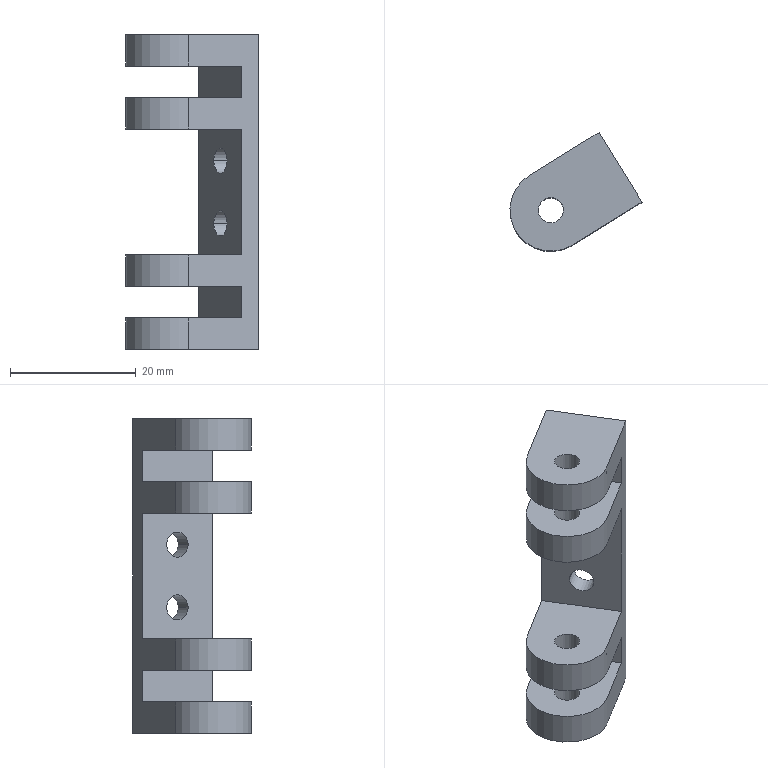Component | SolidWorks | WheelAssembly-1_DamperBase2-1 | 1 solid | 30 faces | box 20.98 x 18.86 x 50 mm | volume 5551 mm3 | cylinder 16 | plane 14 | commonest cylinder face diameters 4 x12 13 x4
build123d program:
from build123d import *

# Parameters (mm, degrees)
SKETCH1_W               = 8
SKETCH1_H               = 8
BOSS_EXTRUDE1_DEPTH     = 42.5
SKETCH2_R               = 2
BOSS_EXTRUDE2_DEPTH     = 25
CUT_EXTRUDE1_DEPTH      = 49.34
CUT_EXTRUDE1_DEPTH_BACK = 49.34
SKETCH3_W               = 5
SKETCH3_H               = 17.65
SKETCH3_W_2             = 20
SKETCH3_H_2             = 17.022
SKETCH4_W               = 50.884
SKETCH4_H               = 95.935
CUT_EXTRUDE2_DEPTH      = 10
SKETCH5_W               = 13
SKETCH5_H               = 50
SKETCH5_R               = 2
BOSS_EXTRUDE3_DEPTH     = 3


with BuildPart() as part:
    # Sketch1 → Boss-Extrude1 (new, symmetric)
    with BuildSketch(Plane.XY):
        Rectangle(SKETCH1_W, SKETCH1_H)
    extrude(amount=BOSS_EXTRUDE1_DEPTH, both=True)

    # Sketch2 → Boss-Extrude2 (add, symmetric)
    with BuildSketch(Plane.XY):
        with BuildLine():
            Line((-6.5, -14), (-6.5, -4))
            Line((-6.5, -4), (6.5, -4))
            Line((6.5, -4), (6.5, -14))
            ThreePointArc((6.5, -14), (0, -20.5), (-6.5, -14))
        make_face()
        with Locations((0, -14)):
            Circle(SKETCH2_R, mode=Mode.SUBTRACT)
    extrude(amount=BOSS_EXTRUDE2_DEPTH, both=True)

    # Sketch3 → Cut-Extrude1 (cut, two sides: drawn at the far end of the back side and taken through both)
    with BuildSketch(Plane(origin=(4, 0, 0), x_dir=(0, 0, -1), z_dir=(1, 0, 0)).offset(-CUT_EXTRUDE1_DEPTH_BACK)):
        with Locations((-17.5, -12.825)):
            Rectangle(SKETCH3_W, SKETCH3_H)
        with Locations((17.5, -12.825)):
            Rectangle(SKETCH3_W, SKETCH3_H)
        with Locations((0, -12.511)):
            Rectangle(SKETCH3_W_2, SKETCH3_H_2)
    extrude(amount=CUT_EXTRUDE1_DEPTH + CUT_EXTRUDE1_DEPTH_BACK, mode=Mode.SUBTRACT)

    # Sketch4 → Cut-Extrude2 (cut)
    with BuildSketch(Plane(origin=(0, -4, 0), x_dir=(1, 0, 0), z_dir=(0, 1, 0))):
        with Locations((5.686, 0.729)):
            Rectangle(SKETCH4_W, SKETCH4_H)
    extrude(amount=CUT_EXTRUDE2_DEPTH, mode=Mode.SUBTRACT)


with BuildPart() as cut_extrude2_piece_1:
    # of the separate pieces the step leaves, piece 1, a body of its own (cut_extrude2_pieces)
    add(part.part.solids().sort_by_distance((-6.5, -4, 15))[0])



with BuildPart() as cut_extrude2_piece_2:
    # of the separate pieces the step leaves, piece 2, a body of its own (cut_extrude2_pieces)
    add(part.part.solids().sort_by_distance((-6.5, -4, -20))[0])


with BuildPart() as cut_extrude2_piece_3:
    # of the separate pieces the step leaves, piece 3, a body of its own (cut_extrude2_pieces)
    add(part.part.solids().sort_by_distance((-6.5, -4, 25))[0])


with BuildPart() as cut_extrude2_piece_4:
    # of the separate pieces the step leaves, piece 4, a body of its own (cut_extrude2_pieces)
    add(part.part.solids().sort_by_distance((-6.5, -4, -10))[0])


with BuildPart() as cut_extrude2_piece_1_1:
    add(cut_extrude2_piece_1.part)

    add(cut_extrude2_piece_2.part)  # Boss-Extrude3 merges Cut-Extrude2 piece 2

    add(cut_extrude2_piece_3.part)  # Boss-Extrude3 merges Cut-Extrude2 piece 3

    add(cut_extrude2_piece_4.part)  # Boss-Extrude3 merges Cut-Extrude2 piece 4
    # Sketch5 → Boss-Extrude3 (add)
    with BuildSketch(Plane(origin=(0, -4, 0), x_dir=(1, 0, 0), z_dir=(0, 1, 0))):
        Rectangle(SKETCH5_W, SKETCH5_H)
        with Locations(Location((0, 5, 0), (0, 0, 180))):
            Circle(SKETCH5_R, mode=Mode.SUBTRACT)
        with Locations(Location((0, -5, 0), (0, 0, 180))):
            Circle(SKETCH5_R, mode=Mode.SUBTRACT)
    extrude(amount=BOSS_EXTRUDE3_DEPTH)


solid = cut_extrude2_piece_1_1.part

# Placed as in the assembly
solid = solid.moved(Location((-246.003, -126.197, -542.97), (0, 0, -58.332)))
STEP:
#1=COLOUR_RGB('',0.7922,0.8196,0.9333);
#2=FILL_AREA_STYLE_COLOUR('',#1);
#3=FILL_AREA_STYLE('',(#2));
#4=SURFACE_STYLE_FILL_AREA(#3);
#5=SURFACE_SIDE_STYLE('',(#4));
#6=SURFACE_STYLE_USAGE(.BOTH.,#5);
#7=PRESENTATION_STYLE_ASSIGNMENT((#6));
#8=CARTESIAN_POINT('',(-10.196,-5.191,-20.983));
#9=VERTEX_POINT('',#8);
#10=CARTESIAN_POINT('',(-10.113,-5.325,-20.983));
#11=VERTEX_POINT('',#10);
#12=CARTESIAN_POINT('',(-10.154,-5.258,-20.983));
#13=DIRECTION('',(0.,0.,1.));
#14=DIRECTION('',(0.8511,0.525,0.));
#15=AXIS2_PLACEMENT_3D('',#12,#13,#14);
#16=CIRCLE('',#15,0.07874);
#17=EDGE_CURVE('',#9,#11,#16,.T.);
#18=ORIENTED_EDGE('',*,*,#17,.F.);
#19=CARTESIAN_POINT('',(-10.196,-5.191,-20.786));
#20=VERTEX_POINT('',#19);
#21=CARTESIAN_POINT('',(-10.196,-5.191,-22.361));
#22=DIRECTION('',(0.,0.,1.));
#23=VECTOR('',#22,39.37);
#24=LINE('',#21,#23);
#25=EDGE_CURVE('',#9,#20,#24,.T.);
#26=ORIENTED_EDGE('',*,*,#25,.T.);
#27=CARTESIAN_POINT('',(-10.113,-5.325,-20.786));
#28=VERTEX_POINT('',#27);
#29=CARTESIAN_POINT('',(-10.154,-5.258,-20.786));
#30=DIRECTION('',(-0.,-0.,-1.));
#31=DIRECTION('',(-0.8511,-0.525,0.));
#32=AXIS2_PLACEMENT_3D('',#29,#30,#31);
#33=CIRCLE('',#32,0.07874);
#34=EDGE_CURVE('',#28,#20,#33,.T.);
#35=ORIENTED_EDGE('',*,*,#34,.F.);
#36=CARTESIAN_POINT('',(-10.113,-5.325,-22.361));
#37=DIRECTION('',(0.,0.,1.));
#38=VECTOR('',#37,39.37);
#39=LINE('',#36,#38);
#40=EDGE_CURVE('',#11,#28,#39,.T.);
#41=ORIENTED_EDGE('',*,*,#40,.F.);
#42=EDGE_LOOP('',(#18,#26,#35,#41));
#43=FACE_OUTER_BOUND('',#42,.T.);
#44=CARTESIAN_POINT('',(-10.154,-5.258,-22.361));
#45=DIRECTION('',(0.,0.,1.));
#46=DIRECTION('',(0.525,-0.8511,0.));
#47=AXIS2_PLACEMENT_3D('',#44,#45,#46);
#48=CYLINDRICAL_SURFACE('',#47,0.07874);
#49=ADVANCED_FACE('',(#43),#48,.F.);
#50=CARTESIAN_POINT('',(-10.196,-5.191,-20.589));
#51=VERTEX_POINT('',#50);
#52=CARTESIAN_POINT('',(-10.113,-5.325,-20.589));
#53=VERTEX_POINT('',#52);
#54=CARTESIAN_POINT('',(-10.154,-5.258,-20.589));
#55=DIRECTION('',(0.,0.,1.));
#56=DIRECTION('',(0.8511,0.525,0.));
#57=AXIS2_PLACEMENT_3D('',#54,#55,#56);
#58=CIRCLE('',#57,0.07874);
#59=EDGE_CURVE('',#51,#53,#58,.T.);
#60=ORIENTED_EDGE('',*,*,#59,.F.);
#61=CARTESIAN_POINT('',(-10.196,-5.191,-20.393));
#62=VERTEX_POINT('',#61);
#63=CARTESIAN_POINT('',(-10.196,-5.191,-22.361));
#64=DIRECTION('',(0.,0.,1.));
#65=VECTOR('',#64,39.37);
#66=LINE('',#63,#65);
#67=EDGE_CURVE('',#51,#62,#66,.T.);
#68=ORIENTED_EDGE('',*,*,#67,.T.);
#69=CARTESIAN_POINT('',(-10.113,-5.325,-20.393));
#70=VERTEX_POINT('',#69);
#71=CARTESIAN_POINT('',(-10.154,-5.258,-20.393));
#72=DIRECTION('',(-0.,-0.,-1.));
#73=DIRECTION('',(-0.525,0.8511,-0.));
#74=AXIS2_PLACEMENT_3D('',#71,#72,#73);
#75=CIRCLE('',#74,0.07874);
#76=EDGE_CURVE('',#70,#62,#75,.T.);
#77=ORIENTED_EDGE('',*,*,#76,.F.);
#78=CARTESIAN_POINT('',(-10.113,-5.325,-22.361));
#79=DIRECTION('',(0.,0.,1.));
#80=VECTOR('',#79,39.37);
#81=LINE('',#78,#80);
#82=EDGE_CURVE('',#53,#70,#81,.T.);
#83=ORIENTED_EDGE('',*,*,#82,.F.);
#84=EDGE_LOOP('',(#60,#68,#77,#83));
#85=FACE_OUTER_BOUND('',#84,.T.);
#86=CARTESIAN_POINT('',(-10.154,-5.258,-22.361));
#87=DIRECTION('',(0.,0.,1.));
#88=DIRECTION('',(0.525,-0.8511,0.));
#89=AXIS2_PLACEMENT_3D('',#86,#87,#88);
#90=CYLINDRICAL_SURFACE('',#89,0.07874);
#91=ADVANCED_FACE('',(#85),#90,.F.);
#92=CARTESIAN_POINT('',(-10.196,-5.191,-21.967));
#93=VERTEX_POINT('',#92);
#94=CARTESIAN_POINT('',(-10.113,-5.325,-21.967));
#95=VERTEX_POINT('',#94);
#96=CARTESIAN_POINT('',(-10.154,-5.258,-21.967));
#97=DIRECTION('',(0.,0.,1.));
#98=DIRECTION('',(0.8511,0.525,0.));
#99=AXIS2_PLACEMENT_3D('',#96,#97,#98);
#100=CIRCLE('',#99,0.07874);
#101=EDGE_CURVE('',#93,#95,#100,.T.);
#102=ORIENTED_EDGE('',*,*,#101,.F.);
#103=CARTESIAN_POINT('',(-10.196,-5.191,-21.77));
#104=VERTEX_POINT('',#103);
#105=CARTESIAN_POINT('',(-10.196,-5.191,-22.361));
#106=DIRECTION('',(0.,0.,1.));
#107=VECTOR('',#106,39.37);
#108=LINE('',#105,#107);
#109=EDGE_CURVE('',#93,#104,#108,.T.);
#110=ORIENTED_EDGE('',*,*,#109,.T.);
#111=CARTESIAN_POINT('',(-10.113,-5.325,-21.77));
#112=VERTEX_POINT('',#111);
#113=CARTESIAN_POINT('',(-10.154,-5.258,-21.77));
#114=DIRECTION('',(-0.,-0.,-1.));
#115=DIRECTION('',(-0.8511,-0.525,0.));
#116=AXIS2_PLACEMENT_3D('',#113,#114,#115);
#117=CIRCLE('',#116,0.07874);
#118=EDGE_CURVE('',#112,#104,#117,.T.);
#119=ORIENTED_EDGE('',*,*,#118,.F.);
#120=CARTESIAN_POINT('',(-10.113,-5.325,-22.361));
#121=DIRECTION('',(0.,0.,1.));
#122=VECTOR('',#121,39.37);
#123=LINE('',#120,#122);
#124=EDGE_CURVE('',#95,#112,#123,.T.);
#125=ORIENTED_EDGE('',*,*,#124,.F.);
#126=EDGE_LOOP('',(#102,#110,#119,#125));
#127=FACE_OUTER_BOUND('',#126,.T.);
#128=CARTESIAN_POINT('',(-10.154,-5.258,-22.361));
#129=DIRECTION('',(0.,0.,1.));
#130=DIRECTION('',(0.525,-0.8511,0.));
#131=AXIS2_PLACEMENT_3D('',#128,#129,#130);
#132=CYLINDRICAL_SURFACE('',#131,0.07874);
#133=ADVANCED_FACE('',(#127),#132,.F.);
#134=CARTESIAN_POINT('',(-9.76,-4.922,-21.574));
#135=VERTEX_POINT('',#134);
#136=CARTESIAN_POINT('',(-9.677,-5.056,-21.574));
#137=VERTEX_POINT('',#136);
#138=CARTESIAN_POINT('',(-9.719,-4.989,-21.574));
#139=DIRECTION('',(0.8511,0.525,-0.));
#140=DIRECTION('',(0.525,-0.8511,0.));
#141=AXIS2_PLACEMENT_3D('',#138,#139,#140);
#142=CIRCLE('',#141,0.07874);
#143=EDGE_CURVE('',#135,#137,#142,.T.);
#144=ORIENTED_EDGE('',*,*,#143,.T.);
#145=CARTESIAN_POINT('',(-9.778,-5.118,-21.574));
#146=VERTEX_POINT('',#145);
#147=CARTESIAN_POINT('',(-9.677,-5.056,-21.574));
#148=DIRECTION('',(-0.8511,-0.525,0.));
#149=VECTOR('',#148,39.37);
#150=LINE('',#147,#149);
#151=EDGE_CURVE('',#137,#146,#150,.T.);
#152=ORIENTED_EDGE('',*,*,#151,.T.);
#153=CARTESIAN_POINT('',(-9.861,-4.984,-21.574));
#154=VERTEX_POINT('',#153);
#155=CARTESIAN_POINT('',(-9.819,-5.051,-21.574));
#156=DIRECTION('',(0.8511,0.525,-0.));
#157=DIRECTION('',(0.525,-0.8511,0.));
#158=AXIS2_PLACEMENT_3D('',#155,#156,#157);
#159=CIRCLE('',#158,0.07874);
#160=EDGE_CURVE('',#154,#146,#159,.T.);
#161=ORIENTED_EDGE('',*,*,#160,.F.);
#162=CARTESIAN_POINT('',(-9.76,-4.922,-21.574));
#163=DIRECTION('',(-0.8511,-0.525,0.));
#164=VECTOR('',#163,39.37);
#165=LINE('',#162,#164);
#166=EDGE_CURVE('',#135,#154,#165,.T.);
#167=ORIENTED_EDGE('',*,*,#166,.F.);
#168=EDGE_LOOP('',(#144,#152,#161,#167));
#169=FACE_OUTER_BOUND('',#168,.T.);
#170=CARTESIAN_POINT('',(-9.719,-4.989,-21.574));
#171=DIRECTION('',(-0.8511,-0.525,0.));
#172=DIRECTION('',(-0.525,0.8511,-0.));
#173=AXIS2_PLACEMENT_3D('',#170,#171,#172);
#174=CYLINDRICAL_SURFACE('',#173,0.07874);
#175=ADVANCED_FACE('',(#169),#174,.F.);
#176=CARTESIAN_POINT('',(-9.76,-4.922,-21.18));
#177=VERTEX_POINT('',#176);
#178=CARTESIAN_POINT('',(-9.677,-5.056,-21.18));
#179=VERTEX_POINT('',#178);
#180=CARTESIAN_POINT('',(-9.719,-4.989,-21.18));
#181=DIRECTION('',(0.8511,0.525,-0.));
#182=DIRECTION('',(0.525,-0.8511,0.));
#183=AXIS2_PLACEMENT_3D('',#180,#181,#182);
#184=CIRCLE('',#183,0.07874);
#185=EDGE_CURVE('',#177,#179,#184,.T.);
#186=ORIENTED_EDGE('',*,*,#185,.T.);
#187=CARTESIAN_POINT('',(-9.778,-5.118,-21.18));
#188=VERTEX_POINT('',#187);
#189=CARTESIAN_POINT('',(-9.677,-5.056,-21.18));
#190=DIRECTION('',(-0.8511,-0.525,0.));
#191=VECTOR('',#190,39.37);
#192=LINE('',#189,#191);
#193=EDGE_CURVE('',#179,#188,#192,.T.);
#194=ORIENTED_EDGE('',*,*,#193,.T.);
#195=CARTESIAN_POINT('',(-9.861,-4.984,-21.18));
#196=VERTEX_POINT('',#195);
#197=CARTESIAN_POINT('',(-9.819,-5.051,-21.18));
#198=DIRECTION('',(0.8511,0.525,-0.));
#199=DIRECTION('',(0.525,-0.8511,0.));
#200=AXIS2_PLACEMENT_3D('',#197,#198,#199);
#201=CIRCLE('',#200,0.07874);
#202=EDGE_CURVE('',#196,#188,#201,.T.);
#203=ORIENTED_EDGE('',*,*,#202,.F.);
#204=CARTESIAN_POINT('',(-9.76,-4.922,-21.18));
#205=DIRECTION('',(-0.8511,-0.525,0.));
#206=VECTOR('',#205,39.37);
#207=LINE('',#204,#206);
#208=EDGE_CURVE('',#177,#196,#207,.T.);
#209=ORIENTED_EDGE('',*,*,#208,.F.);
#210=EDGE_LOOP('',(#186,#194,#203,#209));
#211=FACE_OUTER_BOUND('',#210,.T.);
#212=CARTESIAN_POINT('',(-9.719,-4.989,-21.18));
#213=DIRECTION('',(-0.8511,-0.525,0.));
#214=DIRECTION('',(-0.525,0.8511,-0.));
#215=AXIS2_PLACEMENT_3D('',#212,#213,#214);
#216=CYLINDRICAL_SURFACE('',#215,0.07874);
#217=ADVANCED_FACE('',(#211),#216,.F.);
#218=CARTESIAN_POINT('',(-10.113,-5.325,-22.361));
#219=VERTEX_POINT('',#218);
#220=CARTESIAN_POINT('',(-10.196,-5.191,-22.361));
#221=VERTEX_POINT('',#220);
#222=CARTESIAN_POINT('',(-10.154,-5.258,-22.361));
#223=DIRECTION('',(-0.,-0.,-1.));
#224=DIRECTION('',(-0.525,0.8511,-0.));
#225=AXIS2_PLACEMENT_3D('',#222,#223,#224);
#226=CIRCLE('',#225,0.07874);
#227=EDGE_CURVE('',#219,#221,#226,.T.);
#228=ORIENTED_EDGE('',*,*,#227,.T.);
#229=CARTESIAN_POINT('',(-10.196,-5.191,-22.164));
#230=VERTEX_POINT('',#229);
#231=CARTESIAN_POINT('',(-10.196,-5.191,-22.361));
#232=DIRECTION('',(0.,0.,1.));
#233=VECTOR('',#232,39.37);
#234=LINE('',#231,#233);
#235=EDGE_CURVE('',#221,#230,#234,.T.);
#236=ORIENTED_EDGE('',*,*,#235,.T.);
#237=CARTESIAN_POINT('',(-10.113,-5.325,-22.164));
#238=VERTEX_POINT('',#237);
#239=CARTESIAN_POINT('',(-10.154,-5.258,-22.164));
#240=DIRECTION('',(-0.,-0.,-1.));
#241=DIRECTION('',(-0.8511,-0.525,0.));
#242=AXIS2_PLACEMENT_3D('',#239,#240,#241);
#243=CIRCLE('',#242,0.07874);
#244=EDGE_CURVE('',#238,#230,#243,.T.);
#245=ORIENTED_EDGE('',*,*,#244,.F.);
#246=CARTESIAN_POINT('',(-10.113,-5.325,-22.361));
#247=DIRECTION('',(0.,0.,1.));
#248=VECTOR('',#247,39.37);
#249=LINE('',#246,#248);
#250=EDGE_CURVE('',#219,#238,#249,.T.);
#251=ORIENTED_EDGE('',*,*,#250,.F.);
#252=EDGE_LOOP('',(#228,#236,#245,#251));
#253=FACE_OUTER_BOUND('',#252,.T.);
#254=CARTESIAN_POINT('',(-10.154,-5.258,-22.361));
#255=DIRECTION('',(0.,0.,1.));
#256=DIRECTION('',(0.525,-0.8511,0.));
#257=AXIS2_PLACEMENT_3D('',#254,#255,#256);
#258=CYLINDRICAL_SURFACE('',#257,0.07874);
#259=ADVANCED_FACE('',(#253),#258,.F.);
#260=ORIENTED_EDGE('',*,*,#160,.T.);
#261=CARTESIAN_POINT('',(-9.819,-5.051,-21.574));
#262=DIRECTION('',(0.8511,0.525,-0.));
#263=DIRECTION('',(0.525,-0.8511,0.));
#264=AXIS2_PLACEMENT_3D('',#261,#262,#263);
#265=CIRCLE('',#264,0.07874);
#266=EDGE_CURVE('',#146,#154,#265,.T.);
#267=ORIENTED_EDGE('',*,*,#266,.T.);
#268=EDGE_LOOP('',(#260,#267));
#269=FACE_BOUND('',#268,.T.);
#270=ORIENTED_EDGE('',*,*,#202,.T.);
#271=CARTESIAN_POINT('',(-9.819,-5.051,-21.18));
#272=DIRECTION('',(0.8511,0.525,-0.));
#273=DIRECTION('',(0.525,-0.8511,0.));
#274=AXIS2_PLACEMENT_3D('',#271,#272,#273);
#275=CIRCLE('',#274,0.07874);
#276=EDGE_CURVE('',#188,#196,#275,.T.);
#277=ORIENTED_EDGE('',*,*,#276,.T.);
#278=EDGE_LOOP('',(#270,#277));
#279=FACE_BOUND('',#278,.T.);
#280=CARTESIAN_POINT('',(-9.685,-5.269,-20.983));
#281=VERTEX_POINT('',#280);
#282=CARTESIAN_POINT('',(-9.954,-4.833,-20.983));
#283=VERTEX_POINT('',#282);
#284=CARTESIAN_POINT('',(-9.685,-5.269,-20.983));
#285=DIRECTION('',(-0.525,0.8511,-0.));
#286=VECTOR('',#285,39.37);
#287=LINE('',#284,#286);
#288=EDGE_CURVE('',#281,#283,#287,.T.);
#289=ORIENTED_EDGE('',*,*,#288,.T.);
#290=CARTESIAN_POINT('',(-9.954,-4.833,-21.77));
#291=VERTEX_POINT('',#290);
#292=CARTESIAN_POINT('',(-9.954,-4.833,-20.393));
#293=DIRECTION('',(0.,0.,1.));
#294=VECTOR('',#293,39.37);
#295=LINE('',#292,#294);
#296=EDGE_CURVE('',#291,#283,#295,.T.);
#297=ORIENTED_EDGE('',*,*,#296,.F.);
#298=CARTESIAN_POINT('',(-9.685,-5.269,-21.77));
#299=VERTEX_POINT('',#298);
#300=CARTESIAN_POINT('',(-9.685,-5.269,-21.77));
#301=DIRECTION('',(-0.525,0.8511,-0.));
#302=VECTOR('',#301,39.37);
#303=LINE('',#300,#302);
#304=EDGE_CURVE('',#299,#291,#303,.T.);
#305=ORIENTED_EDGE('',*,*,#304,.F.);
#306=CARTESIAN_POINT('',(-9.685,-5.269,-20.393));
#307=DIRECTION('',(-0.,-0.,-1.));
#308=VECTOR('',#307,39.37);
#309=LINE('',#306,#308);
#310=EDGE_CURVE('',#281,#299,#309,.T.);
#311=ORIENTED_EDGE('',*,*,#310,.F.);
#312=EDGE_LOOP('',(#289,#297,#305,#311));
#313=FACE_OUTER_BOUND('',#312,.T.);
#314=CARTESIAN_POINT('',(-9.819,-5.051,-21.377));
#315=DIRECTION('',(0.8511,0.525,-0.));
#316=DIRECTION('',(-0.,-0.,-1.));
#317=AXIS2_PLACEMENT_3D('',#314,#315,#316);
#318=PLANE('',#317);
#319=ADVANCED_FACE('',(#269,#279,#313),#318,.F.);
#320=CARTESIAN_POINT('',(-9.685,-5.269,-20.786));
#321=VERTEX_POINT('',#320);
#322=CARTESIAN_POINT('',(-9.954,-4.833,-20.786));
#323=VERTEX_POINT('',#322);
#324=CARTESIAN_POINT('',(-9.685,-5.269,-20.786));
#325=DIRECTION('',(-0.525,0.8511,-0.));
#326=VECTOR('',#325,39.37);
#327=LINE('',#324,#326);
#328=EDGE_CURVE('',#321,#323,#327,.T.);
#329=ORIENTED_EDGE('',*,*,#328,.F.);
#330=CARTESIAN_POINT('',(-9.685,-5.269,-20.589));
#331=VERTEX_POINT('',#330);
#332=CARTESIAN_POINT('',(-9.685,-5.269,-20.393));
#333=DIRECTION('',(-0.,-0.,-1.));
#334=VECTOR('',#333,39.37);
#335=LINE('',#332,#334);
#336=EDGE_CURVE('',#331,#321,#335,.T.);
#337=ORIENTED_EDGE('',*,*,#336,.F.);
#338=CARTESIAN_POINT('',(-9.954,-4.833,-20.589));
#339=VERTEX_POINT('',#338);
#340=CARTESIAN_POINT('',(-9.685,-5.269,-20.589));
#341=DIRECTION('',(-0.525,0.8511,-0.));
#342=VECTOR('',#341,39.37);
#343=LINE('',#340,#342);
#344=EDGE_CURVE('',#331,#339,#343,.T.);
#345=ORIENTED_EDGE('',*,*,#344,.T.);
#346=CARTESIAN_POINT('',(-9.954,-4.833,-20.393));
#347=DIRECTION('',(0.,0.,1.));
#348=VECTOR('',#347,39.37);
#349=LINE('',#346,#348);
#350=EDGE_CURVE('',#323,#339,#349,.T.);
#351=ORIENTED_EDGE('',*,*,#350,.F.);
#352=EDGE_LOOP('',(#329,#337,#345,#351));
#353=FACE_OUTER_BOUND('',#352,.T.);
#354=CARTESIAN_POINT('',(-9.819,-5.051,-21.377));
#355=DIRECTION('',(0.8511,0.525,-0.));
#356=DIRECTION('',(-0.,-0.,-1.));
#357=AXIS2_PLACEMENT_3D('',#354,#355,#356);
#358=PLANE('',#357);
#359=ADVANCED_FACE('',(#353),#358,.F.);
#360=CARTESIAN_POINT('',(-9.685,-5.269,-21.967));
#361=VERTEX_POINT('',#360);
#362=CARTESIAN_POINT('',(-9.954,-4.833,-21.967));
#363=VERTEX_POINT('',#362);
#364=CARTESIAN_POINT('',(-9.685,-5.269,-21.967));
#365=DIRECTION('',(-0.525,0.8511,-0.));
#366=VECTOR('',#365,39.37);
#367=LINE('',#364,#366);
#368=EDGE_CURVE('',#361,#363,#367,.T.);
#369=ORIENTED_EDGE('',*,*,#368,.T.);
#370=CARTESIAN_POINT('',(-9.954,-4.833,-22.164));
#371=VERTEX_POINT('',#370);
#372=CARTESIAN_POINT('',(-9.954,-4.833,-20.393));
#373=DIRECTION('',(0.,0.,1.));
#374=VECTOR('',#373,39.37);
#375=LINE('',#372,#374);
#376=EDGE_CURVE('',#371,#363,#375,.T.);
#377=ORIENTED_EDGE('',*,*,#376,.F.);
#378=CARTESIAN_POINT('',(-9.685,-5.269,-22.164));
#379=VERTEX_POINT('',#378);
#380=CARTESIAN_POINT('',(-9.685,-5.269,-22.164));
#381=DIRECTION('',(-0.525,0.8511,-0.));
#382=VECTOR('',#381,39.37);
#383=LINE('',#380,#382);
#384=EDGE_CURVE('',#379,#371,#383,.T.);
#385=ORIENTED_EDGE('',*,*,#384,.F.);
#386=CARTESIAN_POINT('',(-9.685,-5.269,-20.393));
#387=DIRECTION('',(-0.,-0.,-1.));
#388=VECTOR('',#387,39.37);
#389=LINE('',#386,#388);
#390=EDGE_CURVE('',#361,#379,#389,.T.);
#391=ORIENTED_EDGE('',*,*,#390,.F.);
#392=EDGE_LOOP('',(#369,#377,#385,#391));
#393=FACE_OUTER_BOUND('',#392,.T.);
#394=CARTESIAN_POINT('',(-9.819,-5.051,-21.377));
#395=DIRECTION('',(0.8511,0.525,-0.));
#396=DIRECTION('',(-0.,-0.,-1.));
#397=AXIS2_PLACEMENT_3D('',#394,#395,#396);
#398=PLANE('',#397);
#399=ADVANCED_FACE('',(#393),#398,.F.);
#400=CARTESIAN_POINT('',(-10.02,-5.476,-22.361));
#401=VERTEX_POINT('',#400);
#402=CARTESIAN_POINT('',(-10.02,-5.476,-22.164));
#403=VERTEX_POINT('',#402);
#404=CARTESIAN_POINT('',(-10.02,-5.476,-22.361));
#405=DIRECTION('',(0.,0.,1.));
#406=VECTOR('',#405,39.37);
#407=LINE('',#404,#406);
#408=EDGE_CURVE('',#401,#403,#407,.T.);
#409=ORIENTED_EDGE('',*,*,#408,.T.);
#410=CARTESIAN_POINT('',(-10.289,-5.04,-22.164));
#411=VERTEX_POINT('',#410);
#412=CARTESIAN_POINT('',(-10.154,-5.258,-22.164));
#413=DIRECTION('',(-0.,-0.,-1.));
#414=DIRECTION('',(-0.8511,-0.525,0.));
#415=AXIS2_PLACEMENT_3D('',#412,#413,#414);
#416=CIRCLE('',#415,0.2559);
#417=EDGE_CURVE('',#403,#411,#416,.T.);
#418=ORIENTED_EDGE('',*,*,#417,.T.);
#419=CARTESIAN_POINT('',(-10.289,-5.04,-22.361));
#420=VERTEX_POINT('',#419);
#421=CARTESIAN_POINT('',(-10.289,-5.04,-22.361));
#422=DIRECTION('',(0.,0.,1.));
#423=VECTOR('',#422,39.37);
#424=LINE('',#421,#423);
#425=EDGE_CURVE('',#420,#411,#424,.T.);
#426=ORIENTED_EDGE('',*,*,#425,.F.);
#427=CARTESIAN_POINT('',(-10.154,-5.258,-22.361));
#428=DIRECTION('',(-0.,-0.,-1.));
#429=DIRECTION('',(-0.525,0.8511,-0.));
#430=AXIS2_PLACEMENT_3D('',#427,#428,#429);
#431=CIRCLE('',#430,0.2559);
#432=EDGE_CURVE('',#401,#420,#431,.T.);
#433=ORIENTED_EDGE('',*,*,#432,.F.);
#434=EDGE_LOOP('',(#409,#418,#426,#433));
#435=FACE_OUTER_BOUND('',#434,.T.);
#436=CARTESIAN_POINT('',(-10.154,-5.258,-22.361));
#437=DIRECTION('',(0.,0.,1.));
#438=DIRECTION('',(0.525,-0.8511,0.));
#439=AXIS2_PLACEMENT_3D('',#436,#437,#438);
#440=CYLINDRICAL_SURFACE('',#439,0.2559);
#441=ADVANCED_FACE('',(#435),#440,.T.);
#442=ORIENTED_EDGE('',*,*,#425,.T.);
#443=CARTESIAN_POINT('',(-9.954,-4.833,-22.164));
#444=DIRECTION('',(-0.8511,-0.525,0.));
#445=VECTOR('',#444,39.37);
#446=LINE('',#443,#445);
#447=EDGE_CURVE('',#371,#411,#446,.T.);
#448=ORIENTED_EDGE('',*,*,#447,.F.);
#449=ORIENTED_EDGE('',*,*,#376,.T.);
#450=CARTESIAN_POINT('',(-10.289,-5.04,-21.967));
#451=VERTEX_POINT('',#450);
#452=CARTESIAN_POINT('',(-9.954,-4.833,-21.967));
#453=DIRECTION('',(0.8511,0.525,-0.));
#454=VECTOR('',#453,39.37);
#455=LINE('',#452,#454);
#456=EDGE_CURVE('',#451,#363,#455,.T.);
#457=ORIENTED_EDGE('',*,*,#456,.F.);
#458=CARTESIAN_POINT('',(-10.289,-5.04,-21.77));
#459=VERTEX_POINT('',#458);
#460=CARTESIAN_POINT('',(-10.289,-5.04,-22.361));
#461=DIRECTION('',(0.,0.,1.));
#462=VECTOR('',#461,39.37);
#463=LINE('',#460,#462);
#464=EDGE_CURVE('',#451,#459,#463,.T.);
#465=ORIENTED_EDGE('',*,*,#464,.T.);
#466=CARTESIAN_POINT('',(-9.954,-4.833,-21.77));
#467=DIRECTION('',(-0.8511,-0.525,0.));
#468=VECTOR('',#467,39.37);
#469=LINE('',#466,#468);
#470=EDGE_CURVE('',#291,#459,#469,.T.);
#471=ORIENTED_EDGE('',*,*,#470,.F.);
#472=ORIENTED_EDGE('',*,*,#296,.T.);
#473=CARTESIAN_POINT('',(-10.289,-5.04,-20.983));
#474=VERTEX_POINT('',#473);
#475=CARTESIAN_POINT('',(-9.954,-4.833,-20.983));
#476=DIRECTION('',(0.8511,0.525,-0.));
#477=VECTOR('',#476,39.37);
#478=LINE('',#475,#477);
#479=EDGE_CURVE('',#474,#283,#478,.T.);
#480=ORIENTED_EDGE('',*,*,#479,.F.);
#481=CARTESIAN_POINT('',(-10.289,-5.04,-20.786));
#482=VERTEX_POINT('',#481);
#483=CARTESIAN_POINT('',(-10.289,-5.04,-22.361));
#484=DIRECTION('',(0.,0.,1.));
#485=VECTOR('',#484,39.37);
#486=LINE('',#483,#485);
#487=EDGE_CURVE('',#474,#482,#486,.T.);
#488=ORIENTED_EDGE('',*,*,#487,.T.);
#489=CARTESIAN_POINT('',(-9.954,-4.833,-20.786));
#490=DIRECTION('',(-0.8511,-0.525,0.));
#491=VECTOR('',#490,39.37);
#492=LINE('',#489,#491);
#493=EDGE_CURVE('',#323,#482,#492,.T.);
#494=ORIENTED_EDGE('',*,*,#493,.F.);
#495=ORIENTED_EDGE('',*,*,#350,.T.);
#496=CARTESIAN_POINT('',(-10.289,-5.04,-20.589));
#497=VERTEX_POINT('',#496);
#498=CARTESIAN_POINT('',(-9.954,-4.833,-20.589));
#499=DIRECTION('',(0.8511,0.525,-0.));
#500=VECTOR('',#499,39.37);
#501=LINE('',#498,#500);
#502=EDGE_CURVE('',#497,#339,#501,.T.);
#503=ORIENTED_EDGE('',*,*,#502,.F.);
#504=CARTESIAN_POINT('',(-10.289,-5.04,-20.393));
#505=VERTEX_POINT('',#504);
#506=CARTESIAN_POINT('',(-10.289,-5.04,-22.361));
#507=DIRECTION('',(0.,0.,1.));
#508=VECTOR('',#507,39.37);
#509=LINE('',#506,#508);
#510=EDGE_CURVE('',#497,#505,#509,.T.);
#511=ORIENTED_EDGE('',*,*,#510,.T.);
#512=CARTESIAN_POINT('',(-9.853,-4.771,-20.393));
#513=VERTEX_POINT('',#512);
#514=CARTESIAN_POINT('',(-9.853,-4.771,-20.393));
#515=DIRECTION('',(-0.8511,-0.525,0.));
#516=VECTOR('',#515,39.37);
#517=LINE('',#514,#516);
#518=EDGE_CURVE('',#513,#505,#517,.T.);
#519=ORIENTED_EDGE('',*,*,#518,.F.);
#520=CARTESIAN_POINT('',(-9.853,-4.771,-22.361));
#521=VERTEX_POINT('',#520);
#522=CARTESIAN_POINT('',(-9.853,-4.771,-20.393));
#523=DIRECTION('',(0.,0.,1.));
#524=VECTOR('',#523,39.37);
#525=LINE('',#522,#524);
#526=EDGE_CURVE('',#521,#513,#525,.T.);
#527=ORIENTED_EDGE('',*,*,#526,.F.);
#528=CARTESIAN_POINT('',(-9.954,-4.833,-22.361));
#529=DIRECTION('',(0.8511,0.525,-0.));
#530=VECTOR('',#529,39.37);
#531=LINE('',#528,#530);
#532=EDGE_CURVE('',#420,#521,#531,.T.);
#533=ORIENTED_EDGE('',*,*,#532,.F.);
#534=EDGE_LOOP('',(#442,#448,#449,#457,#465,#471,#472,#480,#488,#494,#495,#503,#511,#519,#527,#533));
#535=FACE_OUTER_BOUND('',#534,.T.);
#536=CARTESIAN_POINT('',(-9.954,-4.833,-22.361));
#537=DIRECTION('',(0.525,-0.8511,0.));
#538=DIRECTION('',(-0.8511,-0.525,0.));
#539=AXIS2_PLACEMENT_3D('',#536,#537,#538);
#540=PLANE('',#539);
#541=ADVANCED_FACE('',(#535),#540,.F.);
#542=CARTESIAN_POINT('',(-9.584,-5.207,-22.361));
#543=VERTEX_POINT('',#542);
#544=CARTESIAN_POINT('',(-10.02,-5.476,-22.361));
#545=DIRECTION('',(-0.8511,-0.525,0.));
#546=VECTOR('',#545,39.37);
#547=LINE('',#544,#546);
#548=EDGE_CURVE('',#543,#401,#547,.T.);
#549=ORIENTED_EDGE('',*,*,#548,.F.);
#550=CARTESIAN_POINT('',(-9.584,-5.207,-20.393));
#551=VERTEX_POINT('',#550);
#552=CARTESIAN_POINT('',(-9.584,-5.207,-20.393));
#553=DIRECTION('',(-0.,-0.,-1.));
#554=VECTOR('',#553,39.37);
#555=LINE('',#552,#554);
#556=EDGE_CURVE('',#551,#543,#555,.T.);
#557=ORIENTED_EDGE('',*,*,#556,.F.);
#558=CARTESIAN_POINT('',(-10.02,-5.476,-20.393));
#559=VERTEX_POINT('',#558);
#560=CARTESIAN_POINT('',(-9.584,-5.207,-20.393));
#561=DIRECTION('',(-0.8511,-0.525,0.));
#562=VECTOR('',#561,39.37);
#563=LINE('',#560,#562);
#564=EDGE_CURVE('',#551,#559,#563,.T.);
#565=ORIENTED_EDGE('',*,*,#564,.T.);
#566=CARTESIAN_POINT('',(-10.02,-5.476,-20.589));
#567=VERTEX_POINT('',#566);
#568=CARTESIAN_POINT('',(-10.02,-5.476,-22.361));
#569=DIRECTION('',(0.,0.,1.));
#570=VECTOR('',#569,39.37);
#571=LINE('',#568,#570);
#572=EDGE_CURVE('',#567,#559,#571,.T.);
#573=ORIENTED_EDGE('',*,*,#572,.F.);
#574=CARTESIAN_POINT('',(-9.685,-5.269,-20.589));
#575=DIRECTION('',(0.8511,0.525,-0.));
#576=VECTOR('',#575,39.37);
#577=LINE('',#574,#576);
#578=EDGE_CURVE('',#567,#331,#577,.T.);
#579=ORIENTED_EDGE('',*,*,#578,.T.);
#580=ORIENTED_EDGE('',*,*,#336,.T.);
#581=CARTESIAN_POINT('',(-10.02,-5.476,-20.786));
#582=VERTEX_POINT('',#581);
#583=CARTESIAN_POINT('',(-9.685,-5.269,-20.786));
#584=DIRECTION('',(-0.8511,-0.525,0.));
#585=VECTOR('',#584,39.37);
#586=LINE('',#583,#585);
#587=EDGE_CURVE('',#321,#582,#586,.T.);
#588=ORIENTED_EDGE('',*,*,#587,.T.);
#589=CARTESIAN_POINT('',(-10.02,-5.476,-20.983));
#590=VERTEX_POINT('',#589);
#591=CARTESIAN_POINT('',(-10.02,-5.476,-22.361));
#592=DIRECTION('',(0.,0.,1.));
#593=VECTOR('',#592,39.37);
#594=LINE('',#591,#593);
#595=EDGE_CURVE('',#590,#582,#594,.T.);
#596=ORIENTED_EDGE('',*,*,#595,.F.);
#597=CARTESIAN_POINT('',(-9.685,-5.269,-20.983));
#598=DIRECTION('',(0.8511,0.525,-0.));
#599=VECTOR('',#598,39.37);
#600=LINE('',#597,#599);
#601=EDGE_CURVE('',#590,#281,#600,.T.);
#602=ORIENTED_EDGE('',*,*,#601,.T.);
#603=ORIENTED_EDGE('',*,*,#310,.T.);
#604=CARTESIAN_POINT('',(-10.02,-5.476,-21.77));
#605=VERTEX_POINT('',#604);
#606=CARTESIAN_POINT('',(-9.685,-5.269,-21.77));
#607=DIRECTION('',(-0.8511,-0.525,0.));
#608=VECTOR('',#607,39.37);
#609=LINE('',#606,#608);
#610=EDGE_CURVE('',#299,#605,#609,.T.);
#611=ORIENTED_EDGE('',*,*,#610,.T.);
#612=CARTESIAN_POINT('',(-10.02,-5.476,-21.967));
#613=VERTEX_POINT('',#612);
#614=CARTESIAN_POINT('',(-10.02,-5.476,-22.361));
#615=DIRECTION('',(0.,0.,1.));
#616=VECTOR('',#615,39.37);
#617=LINE('',#614,#616);
#618=EDGE_CURVE('',#613,#605,#617,.T.);
#619=ORIENTED_EDGE('',*,*,#618,.F.);
#620=CARTESIAN_POINT('',(-9.685,-5.269,-21.967));
#621=DIRECTION('',(0.8511,0.525,-0.));
#622=VECTOR('',#621,39.37);
#623=LINE('',#620,#622);
#624=EDGE_CURVE('',#613,#361,#623,.T.);
#625=ORIENTED_EDGE('',*,*,#624,.T.);
#626=ORIENTED_EDGE('',*,*,#390,.T.);
#627=CARTESIAN_POINT('',(-9.685,-5.269,-22.164));
#628=DIRECTION('',(-0.8511,-0.525,0.));
#629=VECTOR('',#628,39.37);
#630=LINE('',#627,#629);
#631=EDGE_CURVE('',#379,#403,#630,.T.);
#632=ORIENTED_EDGE('',*,*,#631,.T.);
#633=ORIENTED_EDGE('',*,*,#408,.F.);
#634=EDGE_LOOP('',(#549,#557,#565,#573,#579,#580,#588,#596,#602,#603,#611,#619,#625,#626,#632,#633));
#635=FACE_OUTER_BOUND('',#634,.T.);
#636=CARTESIAN_POINT('',(-10.02,-5.476,-22.361));
#637=DIRECTION('',(-0.525,0.8511,-0.));
#638=DIRECTION('',(0.,0.,1.));
#639=AXIS2_PLACEMENT_3D('',#636,#637,#638);
#640=PLANE('',#639);
#641=ADVANCED_FACE('',(#635),#640,.F.);
#642=ORIENTED_EDGE('',*,*,#235,.F.);
#643=CARTESIAN_POINT('',(-10.154,-5.258,-22.361));
#644=DIRECTION('',(-0.,-0.,-1.));
#645=DIRECTION('',(-0.525,0.8511,-0.));
#646=AXIS2_PLACEMENT_3D('',#643,#644,#645);
#647=CIRCLE('',#646,0.07874);
#648=EDGE_CURVE('',#221,#219,#647,.T.);
#649=ORIENTED_EDGE('',*,*,#648,.T.);
#650=ORIENTED_EDGE('',*,*,#250,.T.);
#651=CARTESIAN_POINT('',(-10.154,-5.258,-22.164));
#652=DIRECTION('',(-0.,-0.,-1.));
#653=DIRECTION('',(-0.8511,-0.525,0.));
#654=AXIS2_PLACEMENT_3D('',#651,#652,#653);
#655=CIRCLE('',#654,0.07874);
#656=EDGE_CURVE('',#230,#238,#655,.T.);
#657=ORIENTED_EDGE('',*,*,#656,.F.);
#658=EDGE_LOOP('',(#642,#649,#650,#657));
#659=FACE_OUTER_BOUND('',#658,.T.);
#660=CARTESIAN_POINT('',(-10.154,-5.258,-22.361));
#661=DIRECTION('',(0.,0.,1.));
#662=DIRECTION('',(0.525,-0.8511,0.));
#663=AXIS2_PLACEMENT_3D('',#660,#661,#662);
#664=CYLINDRICAL_SURFACE('',#663,0.07874);
#665=ADVANCED_FACE('',(#659),#664,.F.);
#666=ORIENTED_EDGE('',*,*,#432,.T.);
#667=ORIENTED_EDGE('',*,*,#532,.T.);
#668=CARTESIAN_POINT('',(-9.584,-5.207,-22.361));
#669=DIRECTION('',(-0.525,0.8511,-0.));
#670=VECTOR('',#669,39.37);
#671=LINE('',#668,#670);
#672=EDGE_CURVE('',#543,#521,#671,.T.);
#673=ORIENTED_EDGE('',*,*,#672,.F.);
#674=ORIENTED_EDGE('',*,*,#548,.T.);
#675=EDGE_LOOP('',(#666,#667,#673,#674));
#676=FACE_OUTER_BOUND('',#675,.T.);
#677=ORIENTED_EDGE('',*,*,#227,.F.);
#678=ORIENTED_EDGE('',*,*,#648,.F.);
#679=EDGE_LOOP('',(#677,#678));
#680=FACE_BOUND('',#679,.T.);
#681=CARTESIAN_POINT('',(-10.154,-5.258,-22.361));
#682=DIRECTION('',(-0.,-0.,-1.));
#683=DIRECTION('',(-0.525,0.8511,-0.));
#684=AXIS2_PLACEMENT_3D('',#681,#682,#683);
#685=PLANE('',#684);
#686=ADVANCED_FACE('',(#676,#680),#685,.T.);
#687=ORIENTED_EDGE('',*,*,#244,.T.);
#688=ORIENTED_EDGE('',*,*,#656,.T.);
#689=EDGE_LOOP('',(#687,#688));
#690=FACE_BOUND('',#689,.T.);
#691=ORIENTED_EDGE('',*,*,#631,.F.);
#692=ORIENTED_EDGE('',*,*,#384,.T.);
#693=ORIENTED_EDGE('',*,*,#447,.T.);
#694=ORIENTED_EDGE('',*,*,#417,.F.);
#695=EDGE_LOOP('',(#691,#692,#693,#694));
#696=FACE_OUTER_BOUND('',#695,.T.);
#697=CARTESIAN_POINT('',(-9.685,-5.269,-22.164));
#698=DIRECTION('',(-0.,-0.,-1.));
#699=DIRECTION('',(-0.8511,-0.525,0.));
#700=AXIS2_PLACEMENT_3D('',#697,#698,#699);
#701=PLANE('',#700);
#702=ADVANCED_FACE('',(#690,#696),#701,.F.);
#703=ORIENTED_EDGE('',*,*,#185,.F.);
#704=CARTESIAN_POINT('',(-9.719,-4.989,-21.18));
#705=DIRECTION('',(0.8511,0.525,-0.));
#706=DIRECTION('',(0.525,-0.8511,0.));
#707=AXIS2_PLACEMENT_3D('',#704,#705,#706);
#708=CIRCLE('',#707,0.07874);
#709=EDGE_CURVE('',#179,#177,#708,.T.);
#710=ORIENTED_EDGE('',*,*,#709,.F.);
#711=EDGE_LOOP('',(#703,#710));
#712=FACE_BOUND('',#711,.T.);
#713=ORIENTED_EDGE('',*,*,#556,.T.);
#714=ORIENTED_EDGE('',*,*,#672,.T.);
#715=ORIENTED_EDGE('',*,*,#526,.T.);
#716=CARTESIAN_POINT('',(-9.584,-5.207,-20.393));
#717=DIRECTION('',(0.525,-0.8511,0.));
#718=VECTOR('',#717,39.37);
#719=LINE('',#716,#718);
#720=EDGE_CURVE('',#513,#551,#719,.T.);
#721=ORIENTED_EDGE('',*,*,#720,.T.);
#722=EDGE_LOOP('',(#713,#714,#715,#721));
#723=FACE_OUTER_BOUND('',#722,.T.);
#724=ORIENTED_EDGE('',*,*,#143,.F.);
#725=CARTESIAN_POINT('',(-9.719,-4.989,-21.574));
#726=DIRECTION('',(0.8511,0.525,-0.));
#727=DIRECTION('',(0.525,-0.8511,0.));
#728=AXIS2_PLACEMENT_3D('',#725,#726,#727);
#729=CIRCLE('',#728,0.07874);
#730=EDGE_CURVE('',#137,#135,#729,.T.);
#731=ORIENTED_EDGE('',*,*,#730,.F.);
#732=EDGE_LOOP('',(#724,#731));
#733=FACE_BOUND('',#732,.T.);
#734=CARTESIAN_POINT('',(-9.719,-4.989,-21.377));
#735=DIRECTION('',(0.8511,0.525,-0.));
#736=DIRECTION('',(-0.,-0.,-1.));
#737=AXIS2_PLACEMENT_3D('',#734,#735,#736);
#738=PLANE('',#737);
#739=ADVANCED_FACE('',(#712,#723,#733),#738,.T.);
#740=ORIENTED_EDGE('',*,*,#518,.T.);
#741=CARTESIAN_POINT('',(-10.154,-5.258,-20.393));
#742=DIRECTION('',(-0.,-0.,-1.));
#743=DIRECTION('',(-0.525,0.8511,-0.));
#744=AXIS2_PLACEMENT_3D('',#741,#742,#743);
#745=CIRCLE('',#744,0.2559);
#746=EDGE_CURVE('',#559,#505,#745,.T.);
#747=ORIENTED_EDGE('',*,*,#746,.F.);
#748=ORIENTED_EDGE('',*,*,#564,.F.);
#749=ORIENTED_EDGE('',*,*,#720,.F.);
#750=EDGE_LOOP('',(#740,#747,#748,#749));
#751=FACE_OUTER_BOUND('',#750,.T.);
#752=ORIENTED_EDGE('',*,*,#76,.T.);
#753=CARTESIAN_POINT('',(-10.154,-5.258,-20.393));
#754=DIRECTION('',(-0.,-0.,-1.));
#755=DIRECTION('',(-0.525,0.8511,-0.));
#756=AXIS2_PLACEMENT_3D('',#753,#754,#755);
#757=CIRCLE('',#756,0.07874);
#758=EDGE_CURVE('',#62,#70,#757,.T.);
#759=ORIENTED_EDGE('',*,*,#758,.T.);
#760=EDGE_LOOP('',(#752,#759));
#761=FACE_BOUND('',#760,.T.);
#762=CARTESIAN_POINT('',(-9.584,-5.207,-20.393));
#763=DIRECTION('',(-0.,-0.,-1.));
#764=DIRECTION('',(-0.525,0.8511,-0.));
#765=AXIS2_PLACEMENT_3D('',#762,#763,#764);
#766=PLANE('',#765);
#767=ADVANCED_FACE('',(#751,#761),#766,.F.);
#768=ORIENTED_EDGE('',*,*,#193,.F.);
#769=ORIENTED_EDGE('',*,*,#709,.T.);
#770=ORIENTED_EDGE('',*,*,#208,.T.);
#771=ORIENTED_EDGE('',*,*,#276,.F.);
#772=EDGE_LOOP('',(#768,#769,#770,#771));
#773=FACE_OUTER_BOUND('',#772,.T.);
#774=CARTESIAN_POINT('',(-9.719,-4.989,-21.18));
#775=DIRECTION('',(-0.8511,-0.525,0.));
#776=DIRECTION('',(-0.525,0.8511,-0.));
#777=AXIS2_PLACEMENT_3D('',#774,#775,#776);
#778=CYLINDRICAL_SURFACE('',#777,0.07874);
#779=ADVANCED_FACE('',(#773),#778,.F.);
#780=ORIENTED_EDGE('',*,*,#151,.F.);
#781=ORIENTED_EDGE('',*,*,#730,.T.);
#782=ORIENTED_EDGE('',*,*,#166,.T.);
#783=ORIENTED_EDGE('',*,*,#266,.F.);
#784=EDGE_LOOP('',(#780,#781,#782,#783));
#785=FACE_OUTER_BOUND('',#784,.T.);
#786=CARTESIAN_POINT('',(-9.719,-4.989,-21.574));
#787=DIRECTION('',(-0.8511,-0.525,0.));
#788=DIRECTION('',(-0.525,0.8511,-0.));
#789=AXIS2_PLACEMENT_3D('',#786,#787,#788);
#790=CYLINDRICAL_SURFACE('',#789,0.07874);
#791=ADVANCED_FACE('',(#785),#790,.F.);
#792=ORIENTED_EDGE('',*,*,#464,.F.);
#793=CARTESIAN_POINT('',(-10.154,-5.258,-21.967));
#794=DIRECTION('',(0.,0.,1.));
#795=DIRECTION('',(0.8511,0.525,-0.));
#796=AXIS2_PLACEMENT_3D('',#793,#794,#795);
#797=CIRCLE('',#796,0.2559);
#798=EDGE_CURVE('',#451,#613,#797,.T.);
#799=ORIENTED_EDGE('',*,*,#798,.T.);
#800=ORIENTED_EDGE('',*,*,#618,.T.);
#801=CARTESIAN_POINT('',(-10.154,-5.258,-21.77));
#802=DIRECTION('',(-0.,-0.,-1.));
#803=DIRECTION('',(-0.8511,-0.525,0.));
#804=AXIS2_PLACEMENT_3D('',#801,#802,#803);
#805=CIRCLE('',#804,0.2559);
#806=EDGE_CURVE('',#605,#459,#805,.T.);
#807=ORIENTED_EDGE('',*,*,#806,.T.);
#808=EDGE_LOOP('',(#792,#799,#800,#807));
#809=FACE_OUTER_BOUND('',#808,.T.);
#810=CARTESIAN_POINT('',(-10.154,-5.258,-22.361));
#811=DIRECTION('',(0.,0.,1.));
#812=DIRECTION('',(0.525,-0.8511,0.));
#813=AXIS2_PLACEMENT_3D('',#810,#811,#812);
#814=CYLINDRICAL_SURFACE('',#813,0.2559);
#815=ADVANCED_FACE('',(#809),#814,.T.);
#816=ORIENTED_EDGE('',*,*,#109,.F.);
#817=CARTESIAN_POINT('',(-10.154,-5.258,-21.967));
#818=DIRECTION('',(0.,0.,1.));
#819=DIRECTION('',(0.8511,0.525,0.));
#820=AXIS2_PLACEMENT_3D('',#817,#818,#819);
#821=CIRCLE('',#820,0.07874);
#822=EDGE_CURVE('',#95,#93,#821,.T.);
#823=ORIENTED_EDGE('',*,*,#822,.F.);
#824=ORIENTED_EDGE('',*,*,#124,.T.);
#825=CARTESIAN_POINT('',(-10.154,-5.258,-21.77));
#826=DIRECTION('',(-0.,-0.,-1.));
#827=DIRECTION('',(-0.8511,-0.525,0.));
#828=AXIS2_PLACEMENT_3D('',#825,#826,#827);
#829=CIRCLE('',#828,0.07874);
#830=EDGE_CURVE('',#104,#112,#829,.T.);
#831=ORIENTED_EDGE('',*,*,#830,.F.);
#832=EDGE_LOOP('',(#816,#823,#824,#831));
#833=FACE_OUTER_BOUND('',#832,.T.);
#834=CARTESIAN_POINT('',(-10.154,-5.258,-22.361));
#835=DIRECTION('',(0.,0.,1.));
#836=DIRECTION('',(0.525,-0.8511,0.));
#837=AXIS2_PLACEMENT_3D('',#834,#835,#836);
#838=CYLINDRICAL_SURFACE('',#837,0.07874);
#839=ADVANCED_FACE('',(#833),#838,.F.);
#840=ORIENTED_EDGE('',*,*,#118,.T.);
#841=ORIENTED_EDGE('',*,*,#830,.T.);
#842=EDGE_LOOP('',(#840,#841));
#843=FACE_BOUND('',#842,.T.);
#844=ORIENTED_EDGE('',*,*,#610,.F.);
#845=ORIENTED_EDGE('',*,*,#304,.T.);
#846=ORIENTED_EDGE('',*,*,#470,.T.);
#847=ORIENTED_EDGE('',*,*,#806,.F.);
#848=EDGE_LOOP('',(#844,#845,#846,#847));
#849=FACE_OUTER_BOUND('',#848,.T.);
#850=CARTESIAN_POINT('',(-9.685,-5.269,-21.77));
#851=DIRECTION('',(-0.,-0.,-1.));
#852=DIRECTION('',(-0.8511,-0.525,0.));
#853=AXIS2_PLACEMENT_3D('',#850,#851,#852);
#854=PLANE('',#853);
#855=ADVANCED_FACE('',(#843,#849),#854,.F.);
#856=ORIENTED_EDGE('',*,*,#822,.T.);
#857=ORIENTED_EDGE('',*,*,#101,.T.);
#858=EDGE_LOOP('',(#856,#857));
#859=FACE_BOUND('',#858,.T.);
#860=ORIENTED_EDGE('',*,*,#456,.T.);
#861=ORIENTED_EDGE('',*,*,#368,.F.);
#862=ORIENTED_EDGE('',*,*,#624,.F.);
#863=ORIENTED_EDGE('',*,*,#798,.F.);
#864=EDGE_LOOP('',(#860,#861,#862,#863));
#865=FACE_OUTER_BOUND('',#864,.T.);
#866=CARTESIAN_POINT('',(-9.685,-5.269,-21.967));
#867=DIRECTION('',(0.,0.,1.));
#868=DIRECTION('',(0.8511,0.525,-0.));
#869=AXIS2_PLACEMENT_3D('',#866,#867,#868);
#870=PLANE('',#869);
#871=ADVANCED_FACE('',(#859,#865),#870,.F.);
#872=ORIENTED_EDGE('',*,*,#510,.F.);
#873=CARTESIAN_POINT('',(-10.154,-5.258,-20.589));
#874=DIRECTION('',(0.,0.,1.));
#875=DIRECTION('',(0.8511,0.525,-0.));
#876=AXIS2_PLACEMENT_3D('',#873,#874,#875);
#877=CIRCLE('',#876,0.2559);
#878=EDGE_CURVE('',#497,#567,#877,.T.);
#879=ORIENTED_EDGE('',*,*,#878,.T.);
#880=ORIENTED_EDGE('',*,*,#572,.T.);
#881=ORIENTED_EDGE('',*,*,#746,.T.);
#882=EDGE_LOOP('',(#872,#879,#880,#881));
#883=FACE_OUTER_BOUND('',#882,.T.);
#884=CARTESIAN_POINT('',(-10.154,-5.258,-22.361));
#885=DIRECTION('',(0.,0.,1.));
#886=DIRECTION('',(0.525,-0.8511,0.));
#887=AXIS2_PLACEMENT_3D('',#884,#885,#886);
#888=CYLINDRICAL_SURFACE('',#887,0.2559);
#889=ADVANCED_FACE('',(#883),#888,.T.);
#890=ORIENTED_EDGE('',*,*,#67,.F.);
#891=CARTESIAN_POINT('',(-10.154,-5.258,-20.589));
#892=DIRECTION('',(0.,0.,1.));
#893=DIRECTION('',(0.8511,0.525,0.));
#894=AXIS2_PLACEMENT_3D('',#891,#892,#893);
#895=CIRCLE('',#894,0.07874);
#896=EDGE_CURVE('',#53,#51,#895,.T.);
#897=ORIENTED_EDGE('',*,*,#896,.F.);
#898=ORIENTED_EDGE('',*,*,#82,.T.);
#899=ORIENTED_EDGE('',*,*,#758,.F.);
#900=EDGE_LOOP('',(#890,#897,#898,#899));
#901=FACE_OUTER_BOUND('',#900,.T.);
#902=CARTESIAN_POINT('',(-10.154,-5.258,-22.361));
#903=DIRECTION('',(0.,0.,1.));
#904=DIRECTION('',(0.525,-0.8511,0.));
#905=AXIS2_PLACEMENT_3D('',#902,#903,#904);
#906=CYLINDRICAL_SURFACE('',#905,0.07874);
#907=ADVANCED_FACE('',(#901),#906,.F.);
#908=ORIENTED_EDGE('',*,*,#896,.T.);
#909=ORIENTED_EDGE('',*,*,#59,.T.);
#910=EDGE_LOOP('',(#908,#909));
#911=FACE_BOUND('',#910,.T.);
#912=ORIENTED_EDGE('',*,*,#502,.T.);
#913=ORIENTED_EDGE('',*,*,#344,.F.);
#914=ORIENTED_EDGE('',*,*,#578,.F.);
#915=ORIENTED_EDGE('',*,*,#878,.F.);
#916=EDGE_LOOP('',(#912,#913,#914,#915));
#917=FACE_OUTER_BOUND('',#916,.T.);
#918=CARTESIAN_POINT('',(-9.685,-5.269,-20.589));
#919=DIRECTION('',(0.,0.,1.));
#920=DIRECTION('',(0.8511,0.525,-0.));
#921=AXIS2_PLACEMENT_3D('',#918,#919,#920);
#922=PLANE('',#921);
#923=ADVANCED_FACE('',(#911,#917),#922,.F.);
#924=ORIENTED_EDGE('',*,*,#595,.T.);
#925=CARTESIAN_POINT('',(-10.154,-5.258,-20.786));
#926=DIRECTION('',(-0.,-0.,-1.));
#927=DIRECTION('',(-0.8511,-0.525,0.));
#928=AXIS2_PLACEMENT_3D('',#925,#926,#927);
#929=CIRCLE('',#928,0.2559);
#930=EDGE_CURVE('',#582,#482,#929,.T.);
#931=ORIENTED_EDGE('',*,*,#930,.T.);
#932=ORIENTED_EDGE('',*,*,#487,.F.);
#933=CARTESIAN_POINT('',(-10.154,-5.258,-20.983));
#934=DIRECTION('',(0.,0.,1.));
#935=DIRECTION('',(0.8511,0.525,-0.));
#936=AXIS2_PLACEMENT_3D('',#933,#934,#935);
#937=CIRCLE('',#936,0.2559);
#938=EDGE_CURVE('',#474,#590,#937,.T.);
#939=ORIENTED_EDGE('',*,*,#938,.T.);
#940=EDGE_LOOP('',(#924,#931,#932,#939));
#941=FACE_OUTER_BOUND('',#940,.T.);
#942=CARTESIAN_POINT('',(-10.154,-5.258,-22.361));
#943=DIRECTION('',(0.,0.,1.));
#944=DIRECTION('',(0.525,-0.8511,0.));
#945=AXIS2_PLACEMENT_3D('',#942,#943,#944);
#946=CYLINDRICAL_SURFACE('',#945,0.2559);
#947=ADVANCED_FACE('',(#941),#946,.T.);
#948=ORIENTED_EDGE('',*,*,#25,.F.);
#949=CARTESIAN_POINT('',(-10.154,-5.258,-20.983));
#950=DIRECTION('',(0.,0.,1.));
#951=DIRECTION('',(0.8511,0.525,0.));
#952=AXIS2_PLACEMENT_3D('',#949,#950,#951);
#953=CIRCLE('',#952,0.07874);
#954=EDGE_CURVE('',#11,#9,#953,.T.);
#955=ORIENTED_EDGE('',*,*,#954,.F.);
#956=ORIENTED_EDGE('',*,*,#40,.T.);
#957=CARTESIAN_POINT('',(-10.154,-5.258,-20.786));
#958=DIRECTION('',(-0.,-0.,-1.));
#959=DIRECTION('',(-0.8511,-0.525,0.));
#960=AXIS2_PLACEMENT_3D('',#957,#958,#959);
#961=CIRCLE('',#960,0.07874);
#962=EDGE_CURVE('',#20,#28,#961,.T.);
#963=ORIENTED_EDGE('',*,*,#962,.F.);
#964=EDGE_LOOP('',(#948,#955,#956,#963));
#965=FACE_OUTER_BOUND('',#964,.T.);
#966=CARTESIAN_POINT('',(-10.154,-5.258,-22.361));
#967=DIRECTION('',(0.,0.,1.));
#968=DIRECTION('',(0.525,-0.8511,0.));
#969=AXIS2_PLACEMENT_3D('',#966,#967,#968);
#970=CYLINDRICAL_SURFACE('',#969,0.07874);
#971=ADVANCED_FACE('',(#965),#970,.F.);
#972=ORIENTED_EDGE('',*,*,#954,.T.);
#973=ORIENTED_EDGE('',*,*,#17,.T.);
#974=EDGE_LOOP('',(#972,#973));
#975=FACE_BOUND('',#974,.T.);
#976=ORIENTED_EDGE('',*,*,#479,.T.);
#977=ORIENTED_EDGE('',*,*,#288,.F.);
#978=ORIENTED_EDGE('',*,*,#601,.F.);
#979=ORIENTED_EDGE('',*,*,#938,.F.);
#980=EDGE_LOOP('',(#976,#977,#978,#979));
#981=FACE_OUTER_BOUND('',#980,.T.);
#982=CARTESIAN_POINT('',(-9.685,-5.269,-20.983));
#983=DIRECTION('',(0.,0.,1.));
#984=DIRECTION('',(0.8511,0.525,-0.));
#985=AXIS2_PLACEMENT_3D('',#982,#983,#984);
#986=PLANE('',#985);
#987=ADVANCED_FACE('',(#975,#981),#986,.F.);
#988=ORIENTED_EDGE('',*,*,#34,.T.);
#989=ORIENTED_EDGE('',*,*,#962,.T.);
#990=EDGE_LOOP('',(#988,#989));
#991=FACE_BOUND('',#990,.T.);
#992=ORIENTED_EDGE('',*,*,#587,.F.);
#993=ORIENTED_EDGE('',*,*,#328,.T.);
#994=ORIENTED_EDGE('',*,*,#493,.T.);
#995=ORIENTED_EDGE('',*,*,#930,.F.);
#996=EDGE_LOOP('',(#992,#993,#994,#995));
#997=FACE_OUTER_BOUND('',#996,.T.);
#998=CARTESIAN_POINT('',(-9.685,-5.269,-20.786));
#999=DIRECTION('',(-0.,-0.,-1.));
#1000=DIRECTION('',(-0.8511,-0.525,0.));
#1001=AXIS2_PLACEMENT_3D('',#998,#999,#1000);
#1002=PLANE('',#1001);
#1003=ADVANCED_FACE('',(#991,#997),#1002,.F.);
#1004=CLOSED_SHELL('',(#49,#91,#133,#175,#217,#259,#319,#359,#399,#441,#541,#641,#665,#686,#702,#739,#767,#779,#791,#815,#839,#855,#871,#889,#907,#923,#947,#971,#987,#1003));
#1005=MANIFOLD_SOLID_BREP('',#1004);
#1006=STYLED_ITEM('',(#7),#1005);
#1007=(LENGTH_UNIT()NAMED_UNIT(*)SI_UNIT($,.METRE.));
#1008=LENGTH_MEASURE_WITH_UNIT(LENGTH_MEASURE(0.0254),#1007);
#1009=DIMENSIONAL_EXPONENTS(1.,0.,0.,0.,0.,0.,0.);
#1010=(CONVERSION_BASED_UNIT('',#1008)LENGTH_UNIT()NAMED_UNIT(#1009));
#1011=UNCERTAINTY_MEASURE_WITH_UNIT(LENGTH_MEASURE(0.00001),#1010,'','');
#1012=(NAMED_UNIT(*)PLANE_ANGLE_UNIT()SI_UNIT($,.RADIAN.));
#1013=(NAMED_UNIT(*)SI_UNIT($,.STERADIAN.)SOLID_ANGLE_UNIT());
#1014=(GEOMETRIC_REPRESENTATION_CONTEXT(3)GLOBAL_UNCERTAINTY_ASSIGNED_CONTEXT((#1011))GLOBAL_UNIT_ASSIGNED_CONTEXT((#1010,#1012,#1013))REPRESENTATION_CONTEXT('',''));
#1015=MECHANICAL_DESIGN_GEOMETRIC_PRESENTATION_REPRESENTATION('',(#1006),#1014);
#1016=PRESENTATION_LAYER_ASSIGNMENT('','',(#1006));
#1017=CARTESIAN_POINT('',(0.,0.,0.));
#1018=DIRECTION('',(0.,0.,1.));
#1019=DIRECTION('',(1.,0.,0.));
#1020=AXIS2_PLACEMENT_3D('',#1017,#1018,#1019);
#1021=(LENGTH_UNIT()NAMED_UNIT(*)SI_UNIT($,.METRE.));
#1022=LENGTH_MEASURE_WITH_UNIT(LENGTH_MEASURE(0.0254),#1021);
#1023=DIMENSIONAL_EXPONENTS(1.,0.,0.,0.,0.,0.,0.);
#1024=(CONVERSION_BASED_UNIT('',#1022)LENGTH_UNIT()NAMED_UNIT(#1023));
#1025=UNCERTAINTY_MEASURE_WITH_UNIT(LENGTH_MEASURE(0.00001),#1024,'','');
#1026=(NAMED_UNIT(*)PLANE_ANGLE_UNIT()SI_UNIT($,.RADIAN.));
#1027=(NAMED_UNIT(*)SI_UNIT($,.STERADIAN.)SOLID_ANGLE_UNIT());
#1028=(GEOMETRIC_REPRESENTATION_CONTEXT(3)GLOBAL_UNCERTAINTY_ASSIGNED_CONTEXT((#1025))GLOBAL_UNIT_ASSIGNED_CONTEXT((#1024,#1026,#1027))REPRESENTATION_CONTEXT('',''));
#1029=ADVANCED_BREP_SHAPE_REPRESENTATION('',(#1005,#1020),#1028);